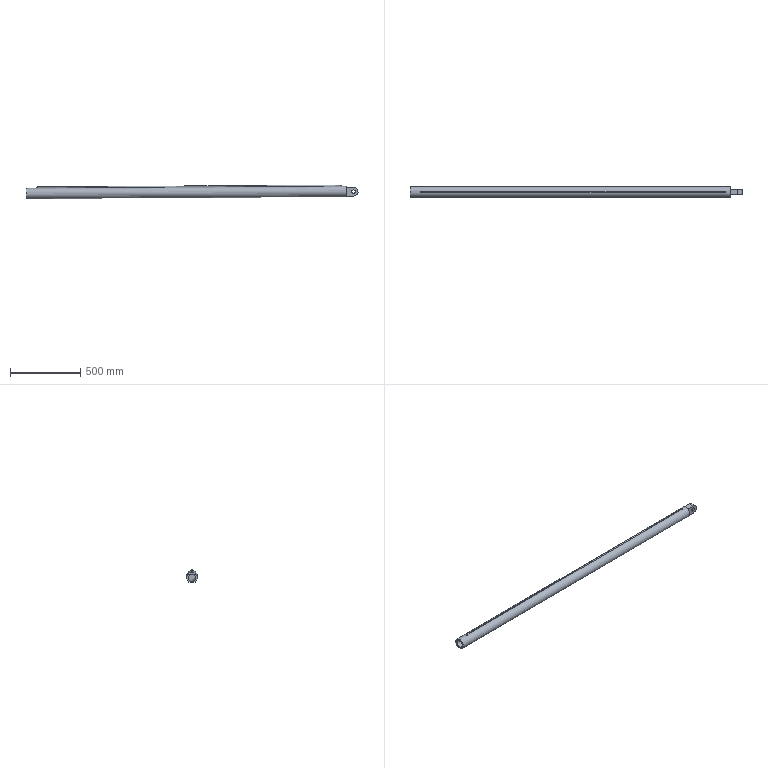Component | NX | CYL_BODY | 2 solids | 18 faces | volume 6013390 mm3 | plane 9 | spline 5 | cylinder 4 | commonest cylinder face diameters 76.2 x1 51 x1 63.5 x1 25.4 x1